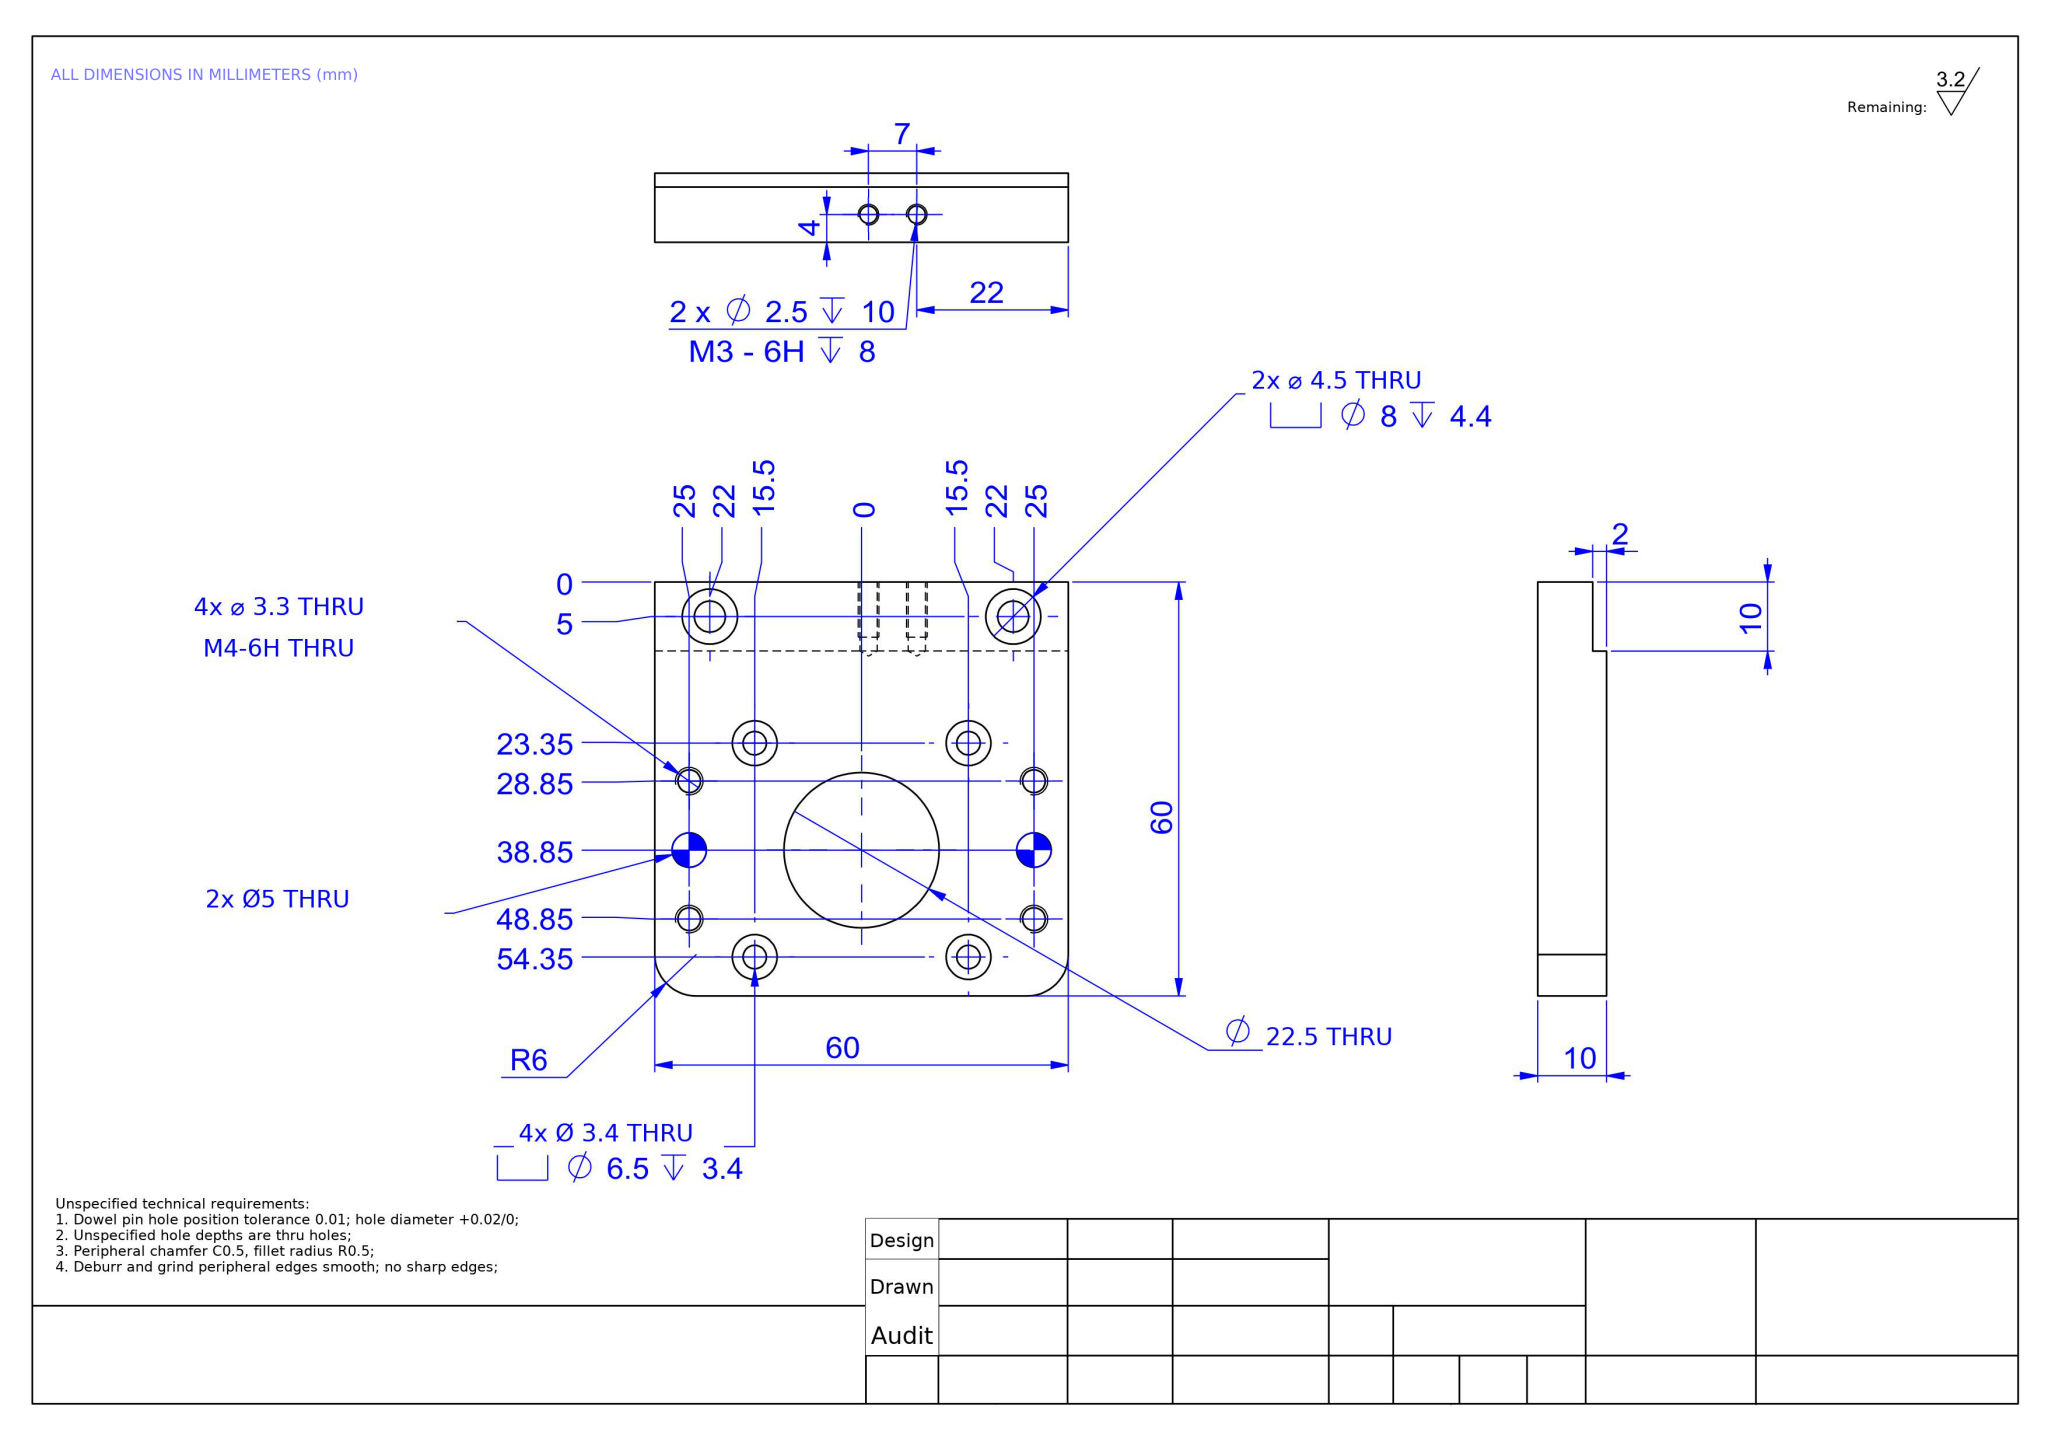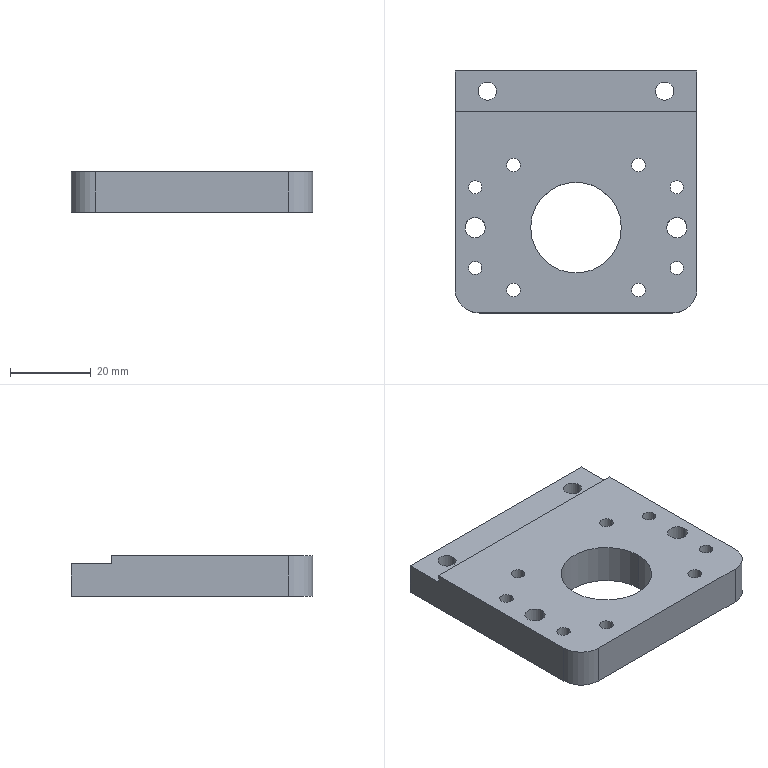Part | NX | mm | 1 solid | 62 faces | box 60 x 60 x 10 mm | volume 28586 mm3 | cylinder 44 | plane 14 | cone 4 | commonest cylinder face diameters 3.3 x8 6.5 x8 3.4 x8 2.5 x4 8 x4 4.5 x4 5 x4 22.5 x2